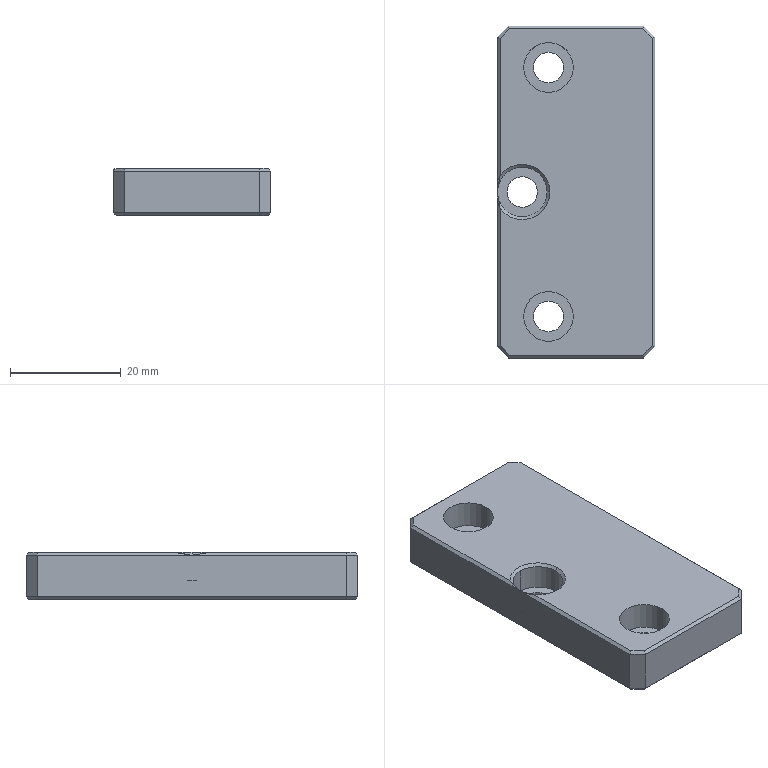CAM job | Mastercam | mm | 4 operations | part box 28.6 x 60 x 8.5
1. Drill/Counterbore | 2 - 6定位倒角
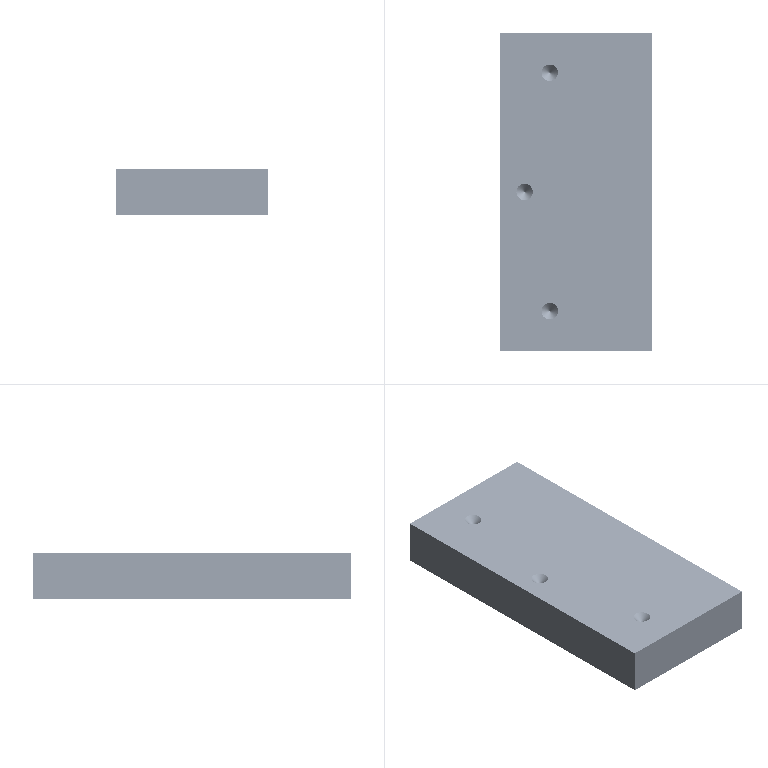2. Peck Drill | 16 - 5.5 钻头
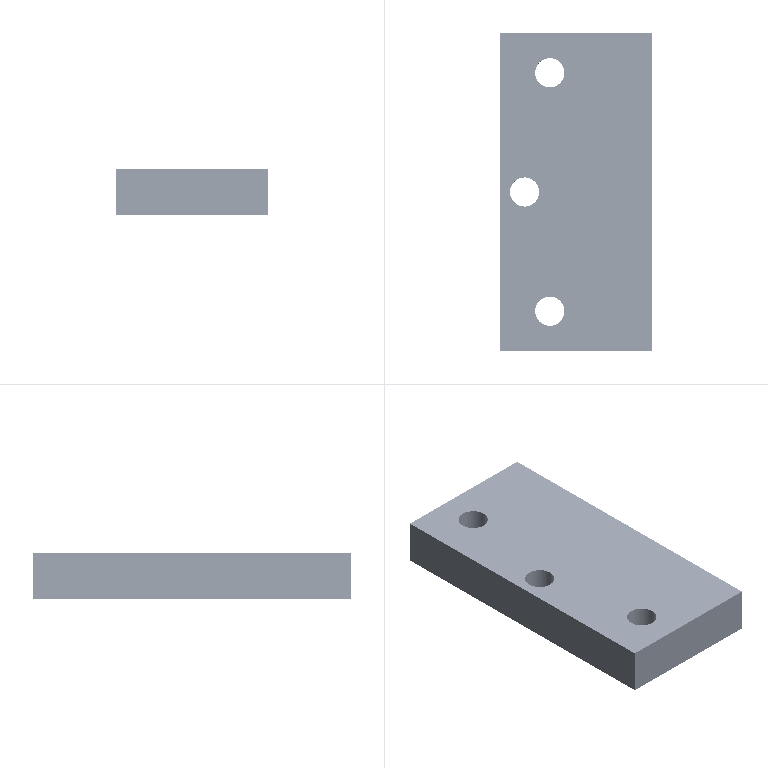3. Helix Bore | 5 - 6 C平底刀
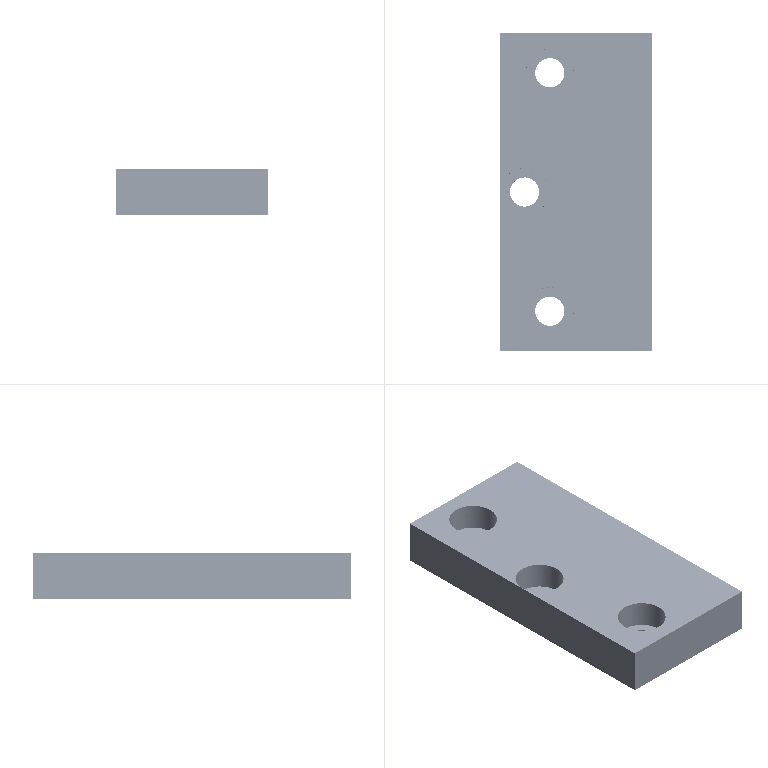4. Contour (2D chamfer) | 2 - 6定位倒角